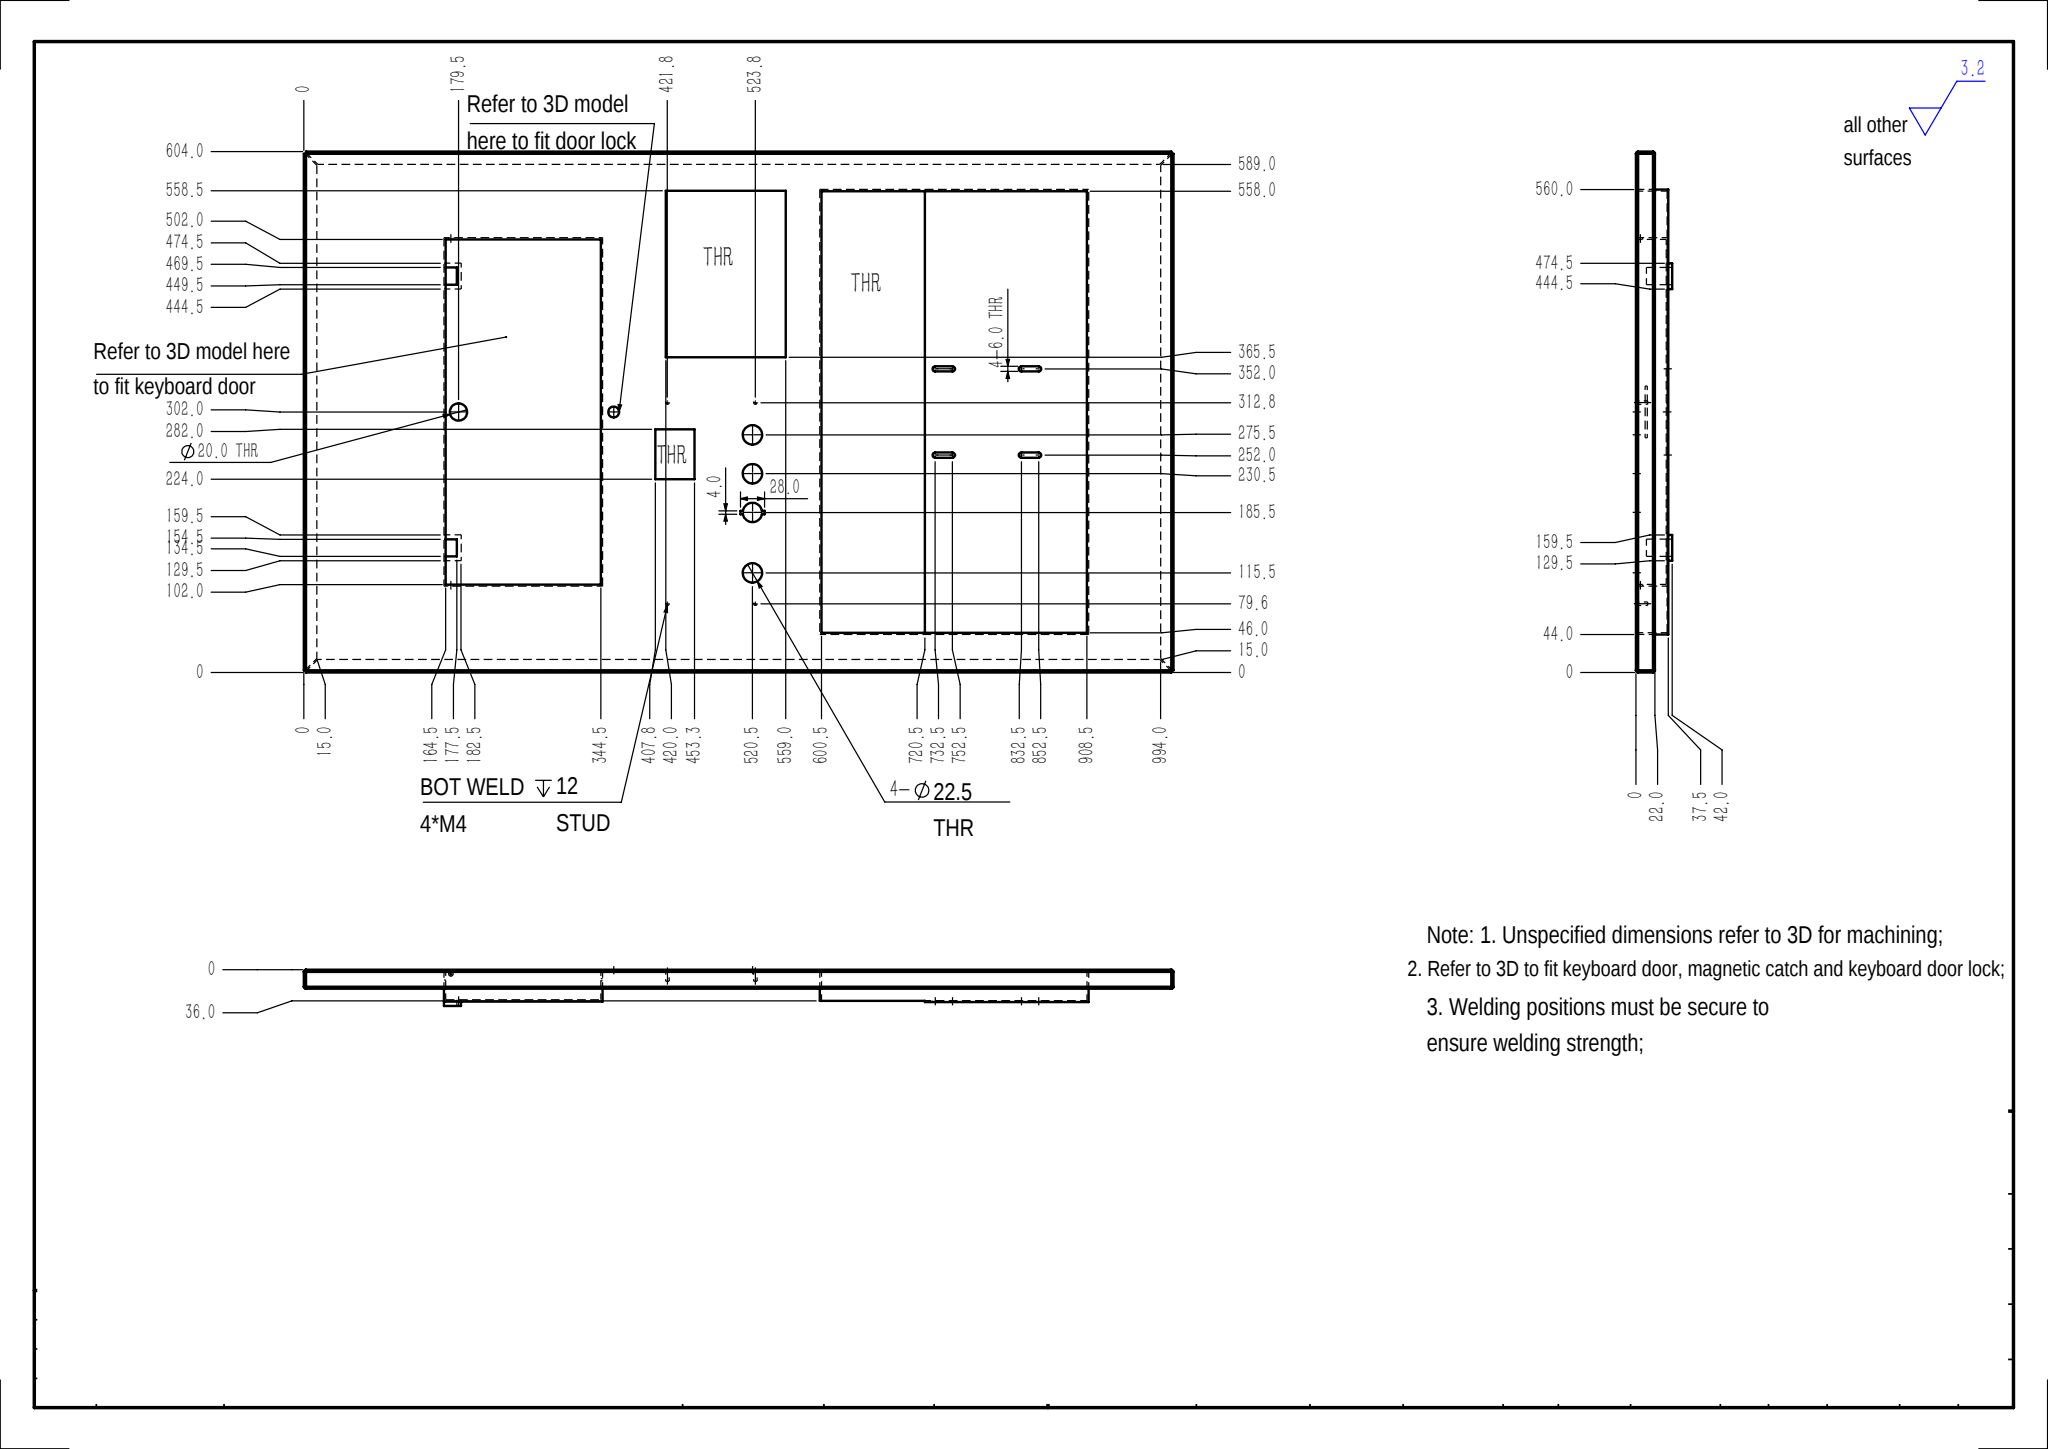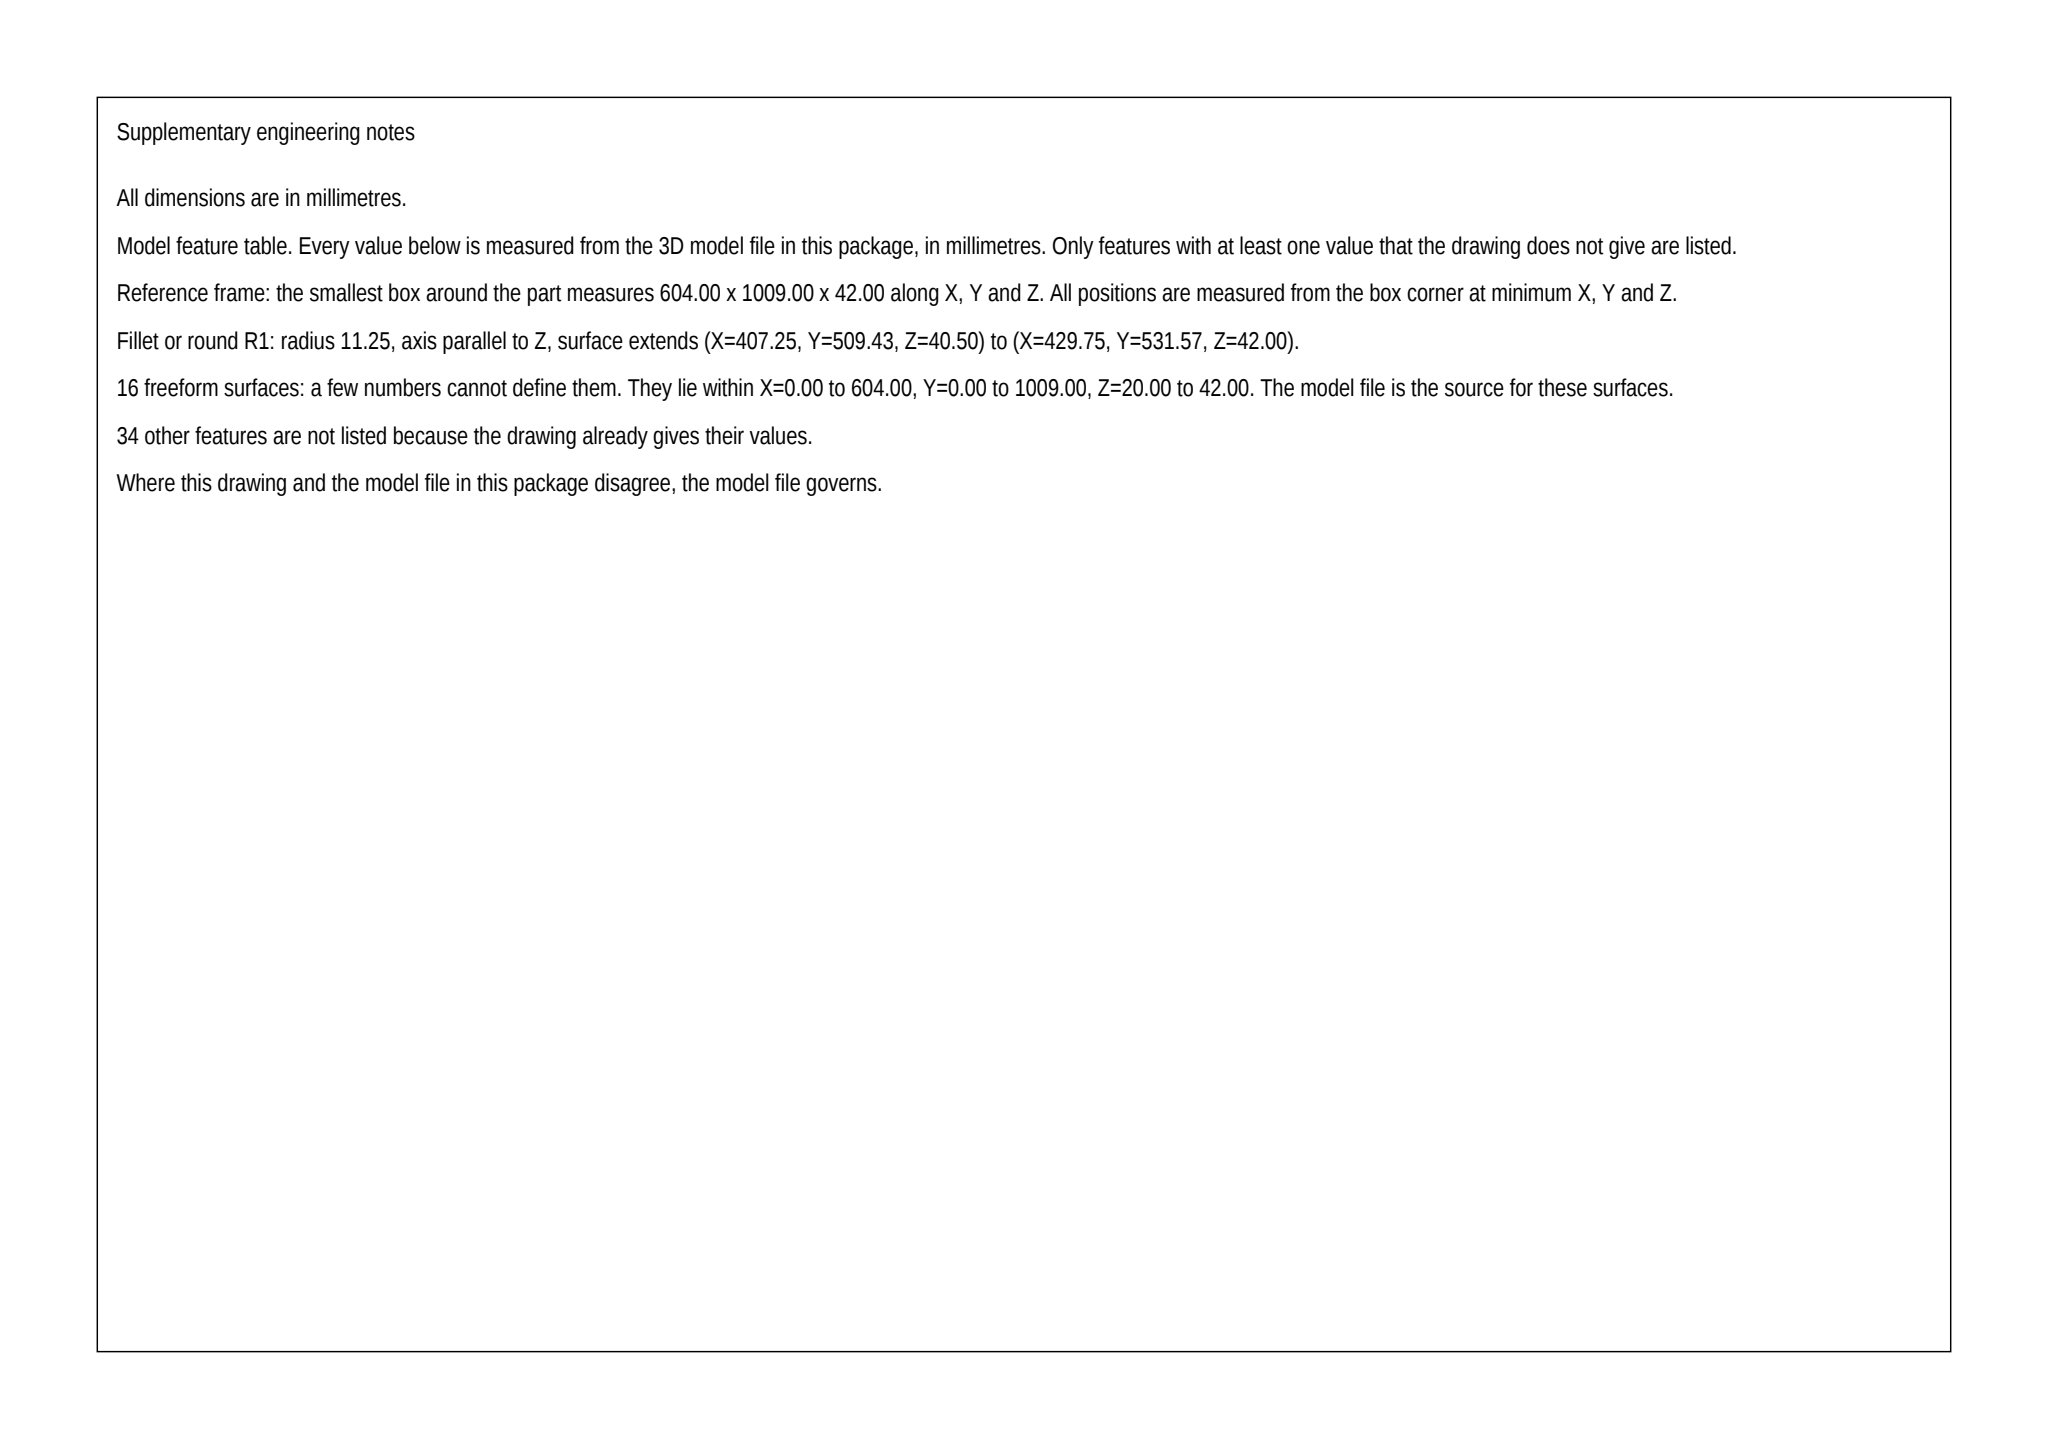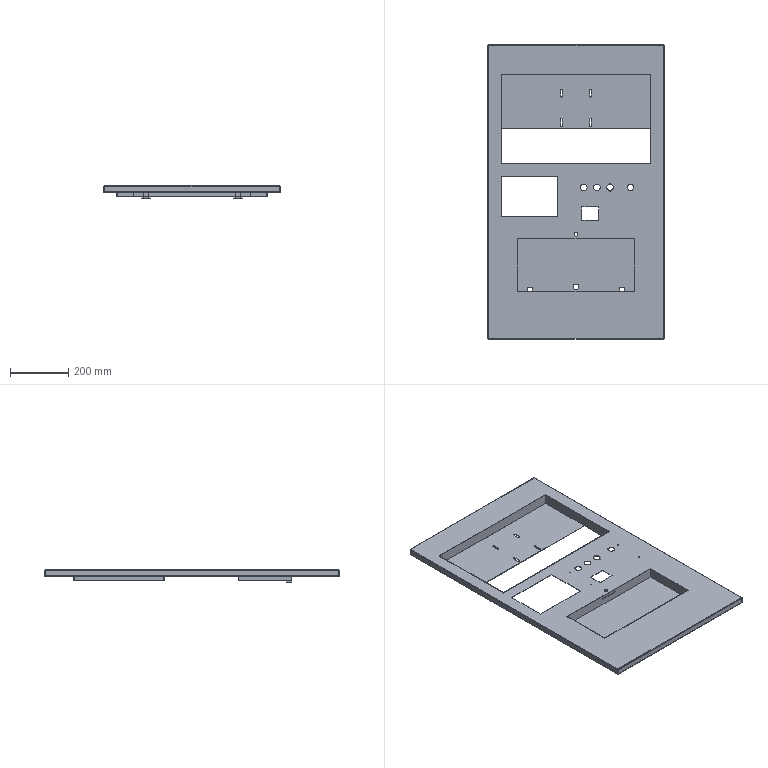Part | SolidWorks | mm | 1 solid | 171 faces | box 604 x 1009 x 42 mm | volume 1164803 mm3 | plane 106 | cylinder 49 | spline 16 | commonest cylinder face diameters 22.5 x9 4 x8 6 x8 5.2 x4 5 x4 2 x4 4.5 x4 1.5 x4
Drawing notes:
Overall length 1009.0 (outer edge to outer edge); existing 994.0 is to inner outline only | from the solid: bbox_xyz y = 1009.03; axis_plane y = 1009.02 vs y = 994.02
Ø12.5 THRU hole at 359.5 from left edge / 302.0 from bottom edge | from the solid: cylinders[12.5,z,[302.02,359.52],count 2]
Lower bracket feature edges located 129.5, 134.5, 154.5 and 159.5 from bottom edge (X datum 0) | from the solid: axis_planes x = 129.52, 134.52, 154.52, 159.52
Step/pocket face levels from back face Z0: 4.5, 5.0, 7.0, 20.0, 21.5, 28.5, 29.0, 30.0, 31.5, 40.5 (overall thickness 42.0) | from the solid: axis_planes z = 4.5, 5.0, 7.0, 20.0, 21.5, 28.5, 29.0, 30.0, 31.5, 40.5, 42.0
Perimeter rolled-edge rounds, all four sides: R0.75 and R2.25 at Z22.25; R1.0 and R2.5 at Z39.5 | from the solid: cylinders dia 1.5 & 4.5 at z 22.25 and dia 2.0 & 5.0 at z 39.5, running full length in x and y
Ø5.2 x 2.0 DEEP holes, axis parallel to the 604 (X) direction, at 170.5 from bottom edge (Y) and 37.0 from back face (Z0): located through the 2.0 thick walls, bores running X=100.0 to 102.0 and X=502.0 to 504.0 from X datum 0. | from the solid: cylinders: hole/bore Ø5.2 axis x at [y=170.5, z=37.0] from 100.0 to 102.0, and from 502.0 to 504.0
Lower raised frame/pocket wall is 2.0 thick: outer faces at X=100.0 and X=504.0 (inner 102.0 / 502.0) and at Y=162.5 and Y=346.5 from bottom edge (inner 164.5 / 344.5). | from the solid: axis_planes: x=100.0 and x=504.0 (extent y 162.5-346.5) vs x=102.0 and x=502.0 (extent y 164.5-344.5); y=162.5 (x 100.0-504.0) vs y=164.5 (x 102.0-502.0); y=344.5 (x 102.0-502.0)
Upper raised frame/pocket wall is 2.0 thick: outer faces at Y=598.5 and Y=910.5 from bottom edge (inner 600.5 / 908.5), between X=44.0 and X=560.0 outer (46.0 / 558.0 inner). | from the solid: axis_planes: x=44.0 and x=560.0 (extent y 598.5-910.5, z 4.5-40.5) vs x=46.0 and x=558.0 (extent y 600.5-908.5, z 6.0-42.0)
4X 45° corner chamfer 12.8 x 12.8, cut in the 1.5 thick perimeter rim/web between Z20.0 and Z21.5 from back face Z0, at the four corners of the rim (X 2.3 / 588.0 to 601.0 and Y 2.3 / 993.0 to 1006.0). | from the solid: inclined_planes: 8 faces at 45.0/45.0/90.0 to XYZ, size 12.8 x 12.8 x 1.5, bbox_from z=20.0 at corners (2.3,3.3), (3.3,2.3), (2.3,993.0), (3.3,994.0), (588.0,2.3), (589.0,3.3), (588.0,994.0)
Perimeter rim/web face level: rim is 1.5 thick, Z20.0 to Z21.5 from back face Z0; rim inner faces at X=15.0 and X=589.0 from bottom edge and Y=15.0 from left edge. | from the solid: axis_planes x=15.0 and x=589.0, extent z [20.0, 21.5]; y=15.0 extent z [20.0, 21.5]
Lower raised frame/pocket (X=100.0/504.0, Y=162.5/346.5): outer wall faces run Z5.0 to Z40.5; inner wall faces (X=102.0/502.0, Y=164.5/344.5) run Z7.0 to Z42.0 from back face Z0. | from the solid: axis_planes x=100.0 & x=504.0 extent z [5.0,40.5]; x=102.0 & x=502.0 and y=164.5 & y=344.5 extent z [7.0,42.0]; y=162.5 extent z [0.0,40.5]
Upper raised frame/pocket (X=44.0/560.0, Y=598.5/910.5): outer wall faces run Z4.5 to Z40.5; inner wall faces (X=46.0/558.0, Y=600.5/908.5) run Z6.0 to Z42.0 from back face Z0. | from the solid: axis_planes x=44.0 & x=560.0 extent z [4.5,40.5]; x=46.0 & x=558.0 extent z [6.0,42.0]
Lower bracket features: the 129.5-to-159.5 and 444.5-to-474.5 (X from bottom edge) faces run Z0 to Z5.0; the 134.5/154.5 and 449.5/469.5 webs run Z0 to Z30.0; bracket ends at Y=177.5 run Z0 to Z7.0 and at Y=182.5 run Z0 to Z5.0 from back face Z0. | from the solid: axis_planes x=129.5/159.5/444.5/474.5 extent z [0.0,5.0]; x=134.5/154.5/449.5/469.5 extent z [0.0,30.0]; y=177.5 extent z [0.0,7.0]; y=182.5 extent z [0.0,5.0]
Central 28.0 wide feature (X=272.0 to 332.0 from bottom edge, Y=344.5 to 346.5 from left edge): face level Z29.0 to Z31.5 from back face Z0. | from the solid: axis_planes x=272.0 and x=332.0, extent y [344.5,346.5], z [29.0,31.5]
4X Ø4.0 boss, 12.0 high, from Z28.5 to Z40.5 from back face Z0, at X=291.2 and 524.4 from bottom edge, Y=421.8 and 523.8 from left edge. | from the solid: cylinders boss/shaft dia 4.0, axis z, at (291.2,421.8), (291.2,523.8), (524.4,421.8), (524.4,523.8), from 28.5 to 40.5
8X Ø6.0 slot-end features break the 1.5 thick wall from Z4.5 to Z6.0 from back face Z0, at X=252.0 and 352.0 from bottom edge, Y=732.5, 752.5, 832.5 and 852.5 from left edge. | from the solid: cylinders dia 6.0 axis z at (252.0/352.0, 732.5/752.5/832.5/852.5), from 4.5 to 6.0
Ø20.0 x 2.0 DEEP blind hole face level: bore runs Z5.0 to Z7.0 from back face Z0 (X=302.0 from bottom edge, Y=179.5 from left edge). | from the solid: cylinders hole/bore dia 20.0 axis z at (302.0,179.5), from 5.0 to 7.0
Ø12.5 THRU and 4X Ø22.5 THRU pierce the 1.5 thick wall from Z40.5 to Z42.0 from back face Z0 (Ø12.5 at X=302.0/Y=359.5; Ø22.5 at Y=520.5, X=328.5, 373.5, 418.5, 488.5). | from the solid: cylinders dia 12.5 at (302.0,359.5) and dia 22.5 at (328.5/373.5/418.5/488.5, 520.5), all from 40.5 to 42.0
Outer perimeter skirt/flange wall 1.5 thick, extending Z22.2 to Z39.5 from back face Z0: side wall outer faces at X=0 and X=604.0, inner faces at X=1.5 and X=602.5 (from X datum 0). | from the solid: axis_planes normal x at offsets 0.0, 1.5, 602.5, 604.0, each extent z=[22.2,39.5], y=[2.6,1006.5]
Outer perimeter skirt/flange end walls 1.5 thick, extending Z22.2 to Z39.5 from back face Z0: outer faces at Y=0 and Y=1009.0, inner faces at Y=1.5 and Y=1007.5 (from left edge datum 0). | from the solid: axis_planes normal y at offsets 0.0, 1.5, 1007.5, 1009.0, each extent z=[22.2,39.5], x=[2.6,601.5]